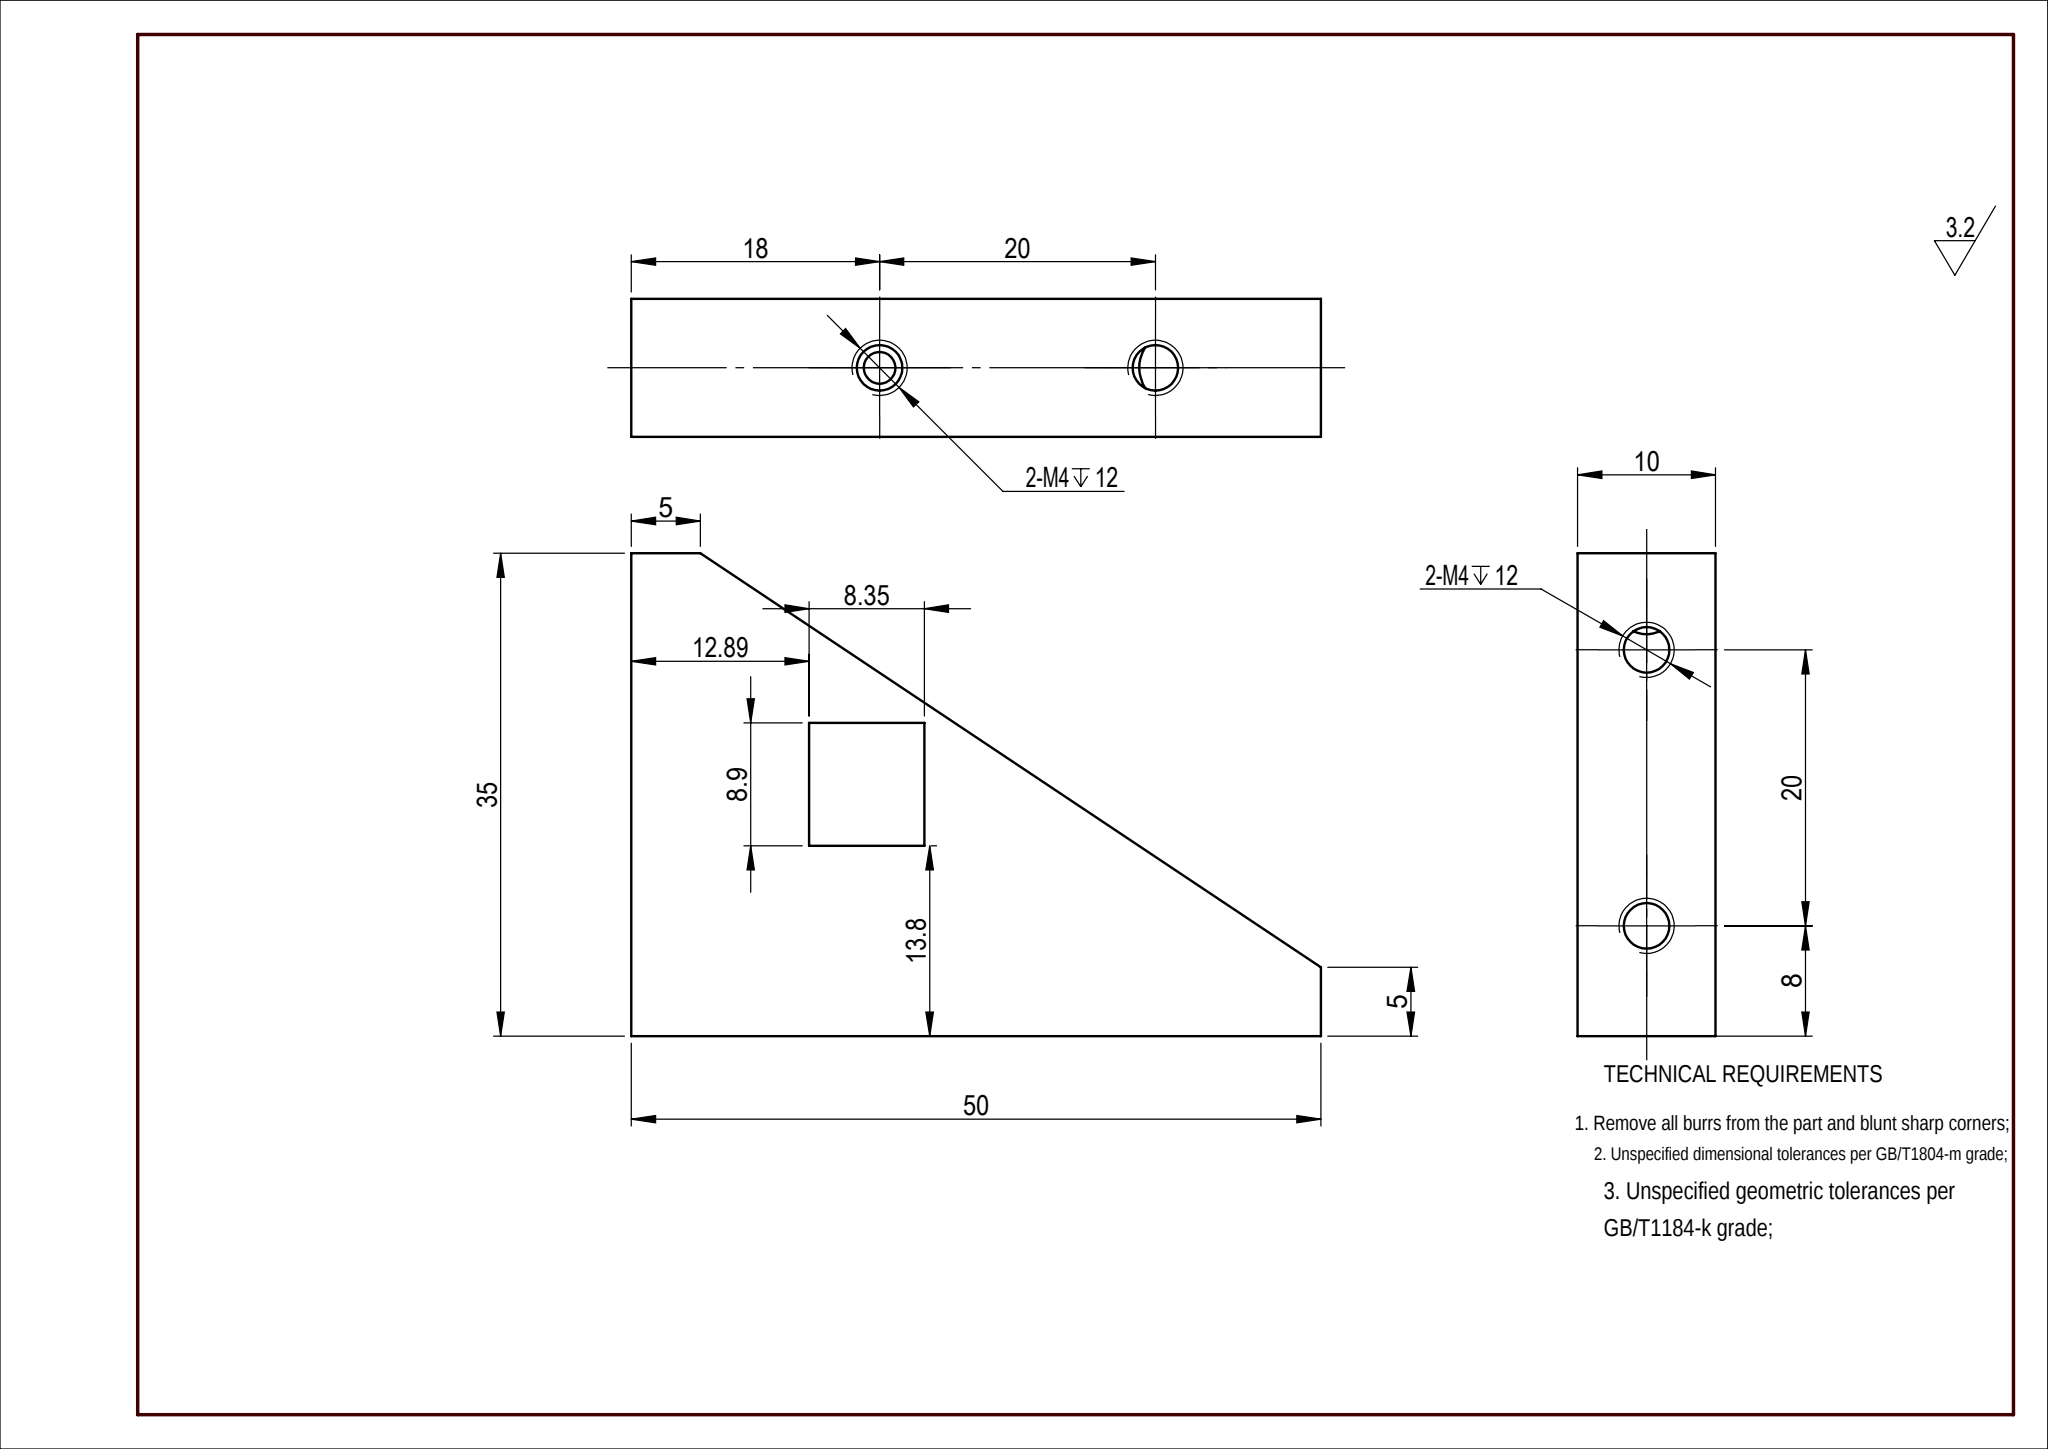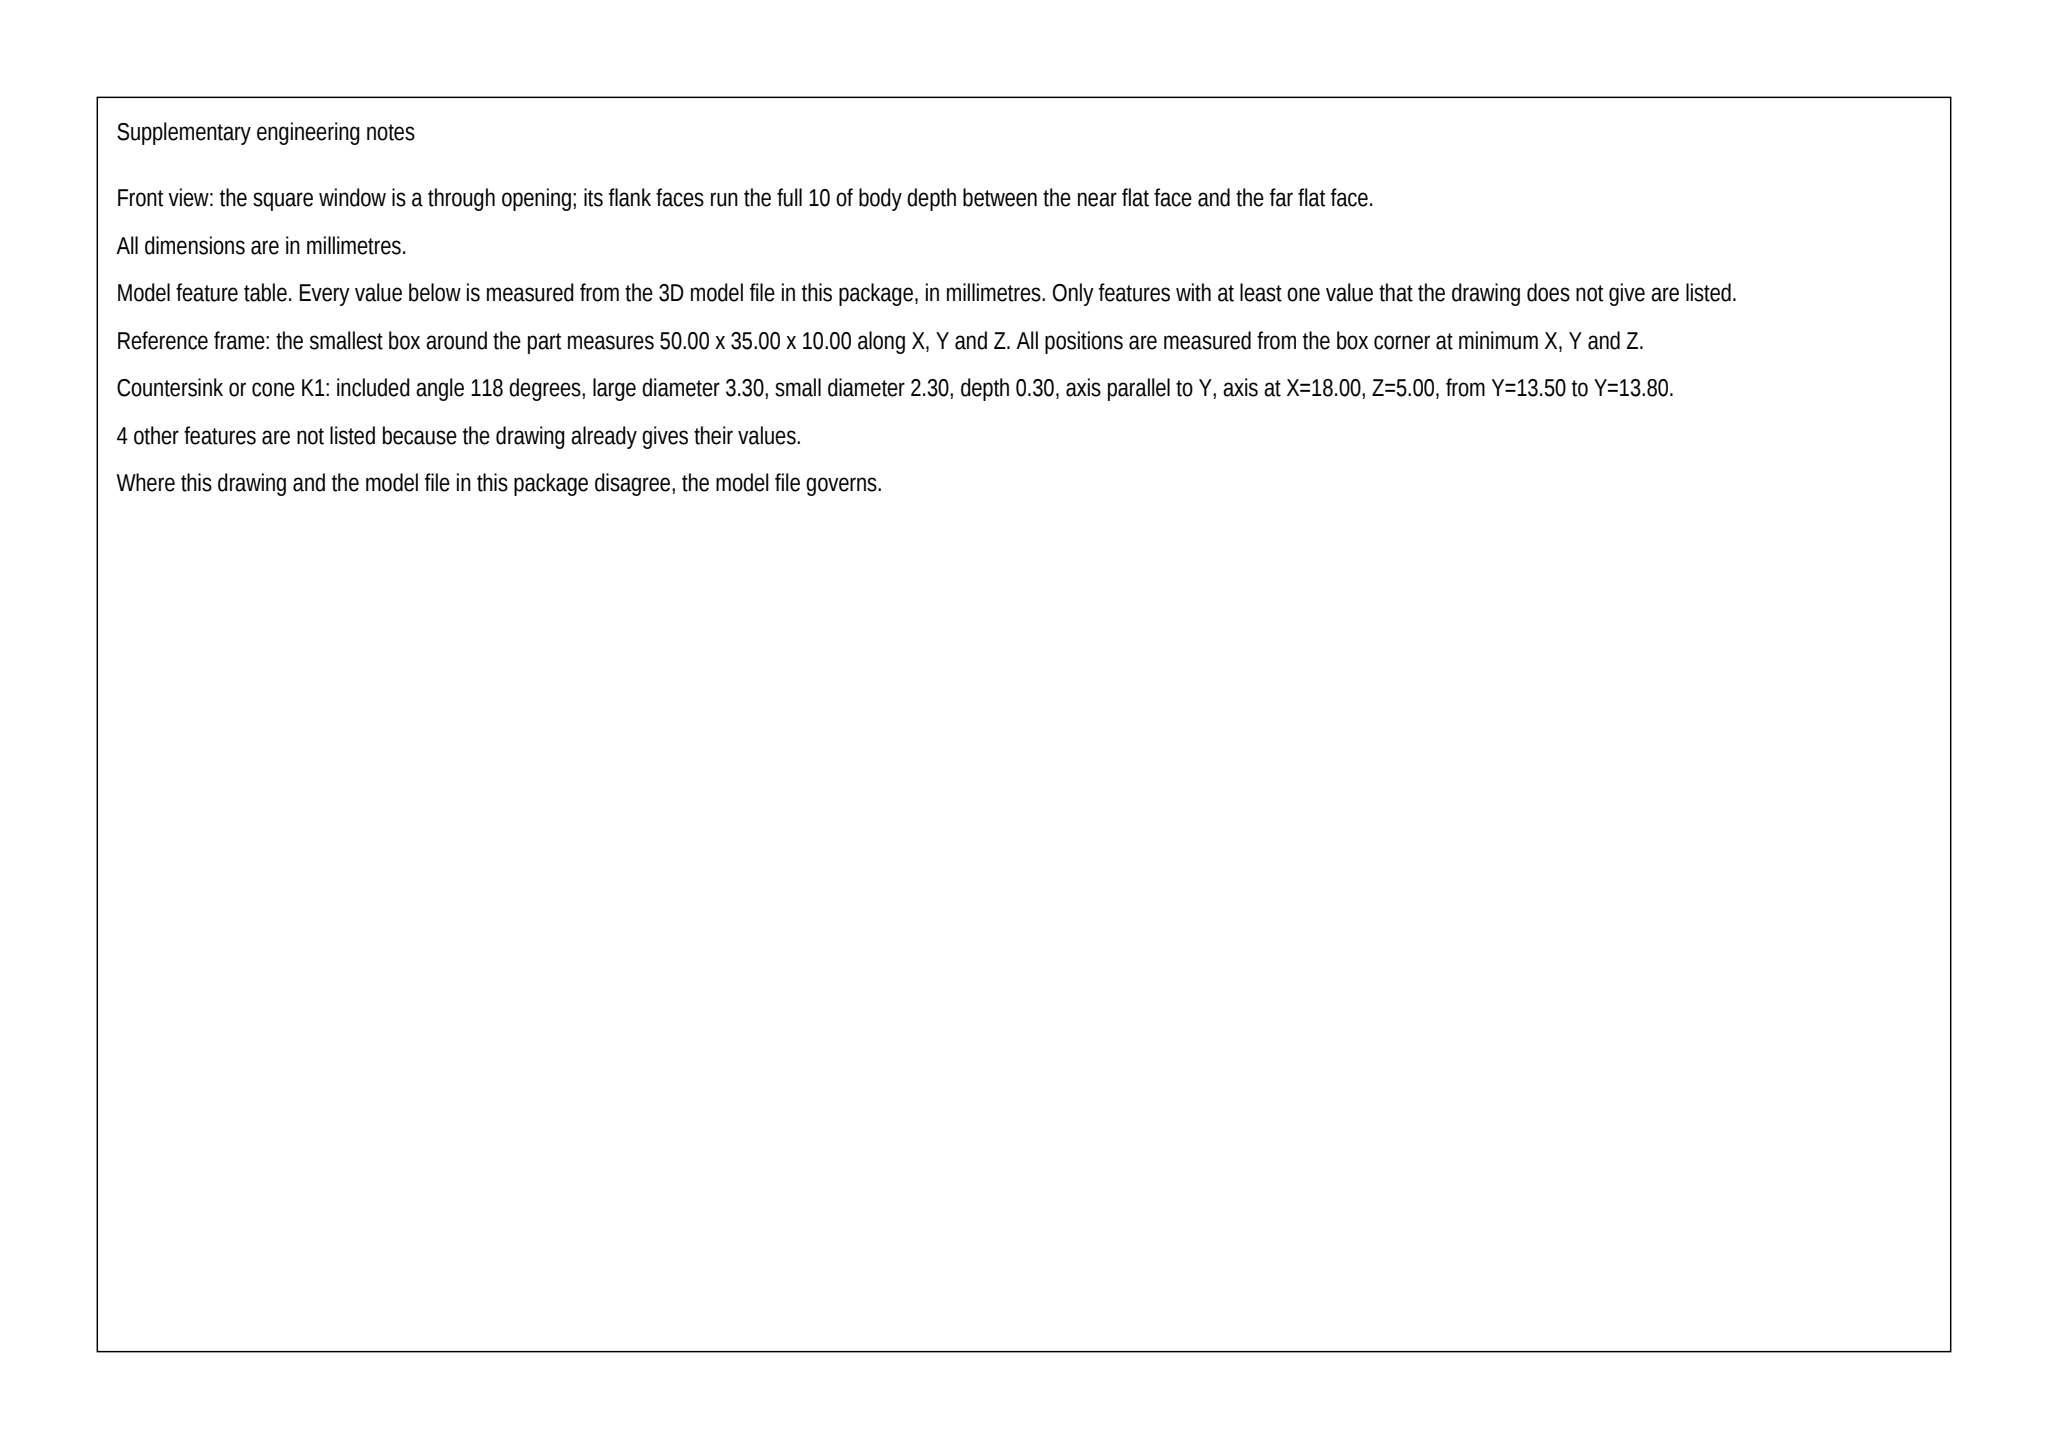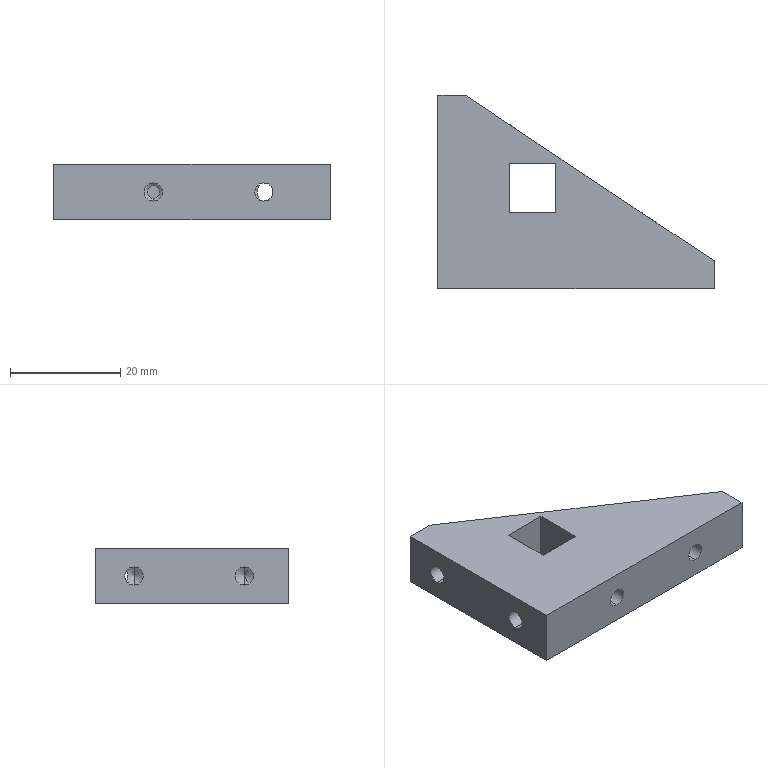Part | SolidWorks | mm | 1 solid | 26 faces | box 50 x 35 x 10 mm | volume 9542 mm3 | plane 11 | cylinder 8 | cone 7 | commonest cylinder face diameters 3.3 x8
build123d program:
from build123d import *

# Parameters (mm, degrees)
BOSS_EXTRUDE1_DEPTH   = 5
M4_TAPPED_HOLE1_D     = 3.3
M4_TAPPED_HOLE1_DEPTH = 13.5
M4_TAPPED_HOLE1_TIP   = 0.9914
M4_TAPPED_HOLE2_D     = 3.3
M4_TAPPED_HOLE2_DEPTH = 13.5
M4_TAPPED_HOLE2_TIP   = 0.9914
SKETCH6_W             = 8.348
SKETCH6_H             = 8.902
CUT_EXTRUDE1_DEPTH    = 22


with BuildPart() as part:
    # Sketch1 → Boss-Extrude1 (new, symmetric)
    with BuildSketch(Plane.XY):
        Polygon((0, 0), (0, 35), (5, 35), (50, 5), (50, 0), align=None)
    extrude(amount=BOSS_EXTRUDE1_DEPTH, both=True)

    # M4 Tapped Hole1
    with Locations(Plane.ZY):
        with Locations((0, 8), (0, 28)):
            Hole(M4_TAPPED_HOLE1_D / 2, depth=M4_TAPPED_HOLE1_DEPTH)
            with Locations((0, 0, -(M4_TAPPED_HOLE1_DEPTH + M4_TAPPED_HOLE1_TIP / 2))):  # 118° drill point
                Cone(0, M4_TAPPED_HOLE1_D / 2, M4_TAPPED_HOLE1_TIP, mode=Mode.SUBTRACT)

    # M4 Tapped Hole2
    with Locations(Plane.XZ):
        with Locations((18, 0), (38, 0)):
            Hole(M4_TAPPED_HOLE2_D / 2, depth=M4_TAPPED_HOLE2_DEPTH)
            with Locations((0, 0, -(M4_TAPPED_HOLE2_DEPTH + M4_TAPPED_HOLE2_TIP / 2))):  # 118° drill point
                Cone(0, M4_TAPPED_HOLE2_D / 2, M4_TAPPED_HOLE2_TIP, mode=Mode.SUBTRACT)

    # Sketch6 → Cut-Extrude1 (cut)
    with BuildSketch(Plane(origin=(0, 0, -5), x_dir=(-1, 0, 0), z_dir=(0, 0, -1))):
        with Locations((-17.067, 18.252)):
            Rectangle(SKETCH6_W, SKETCH6_H)
    extrude(amount=-CUT_EXTRUDE1_DEPTH, mode=Mode.SUBTRACT)


solid = part.part
STEP:
#1=CARTESIAN_POINT('',(18.,13.5,1.65));
#2=VERTEX_POINT('',#1);
#3=CARTESIAN_POINT('',(18.,13.5,-1.65));
#4=VERTEX_POINT('',#3);
#5=CARTESIAN_POINT('',(18.,13.5,0.));
#6=DIRECTION('',(0.,-1.,0.));
#7=DIRECTION('',(0.,0.,-1.));
#8=AXIS2_PLACEMENT_3D('',#5,#6,#7);
#9=CIRCLE('',#8,1.65);
#10=EDGE_CURVE('',#2,#4,#9,.T.);
#11=ORIENTED_EDGE('',*,*,#10,.F.);
#12=CARTESIAN_POINT('',(18.,-0.,1.65));
#13=VERTEX_POINT('',#12);
#14=CARTESIAN_POINT('',(18.,0.,1.65));
#15=DIRECTION('',(0.,-1.,0.));
#16=VECTOR('',#15,1000.);
#17=LINE('',#14,#16);
#18=EDGE_CURVE('',#2,#13,#17,.T.);
#19=ORIENTED_EDGE('',*,*,#18,.T.);
#20=CARTESIAN_POINT('',(18.,-0.,-1.65));
#21=VERTEX_POINT('',#20);
#22=CARTESIAN_POINT('',(18.,-0.,0.));
#23=DIRECTION('',(0.,-1.,0.));
#24=DIRECTION('',(0.,0.,-1.));
#25=AXIS2_PLACEMENT_3D('',#22,#23,#24);
#26=CIRCLE('',#25,1.65);
#27=EDGE_CURVE('',#13,#21,#26,.T.);
#28=ORIENTED_EDGE('',*,*,#27,.T.);
#29=CARTESIAN_POINT('',(18.,0.,-1.65));
#30=DIRECTION('',(0.,-1.,0.));
#31=VECTOR('',#30,1000.);
#32=LINE('',#29,#31);
#33=EDGE_CURVE('',#4,#21,#32,.T.);
#34=ORIENTED_EDGE('',*,*,#33,.F.);
#35=EDGE_LOOP('',(#11,#19,#28,#34));
#36=FACE_OUTER_BOUND('',#35,.T.);
#37=CARTESIAN_POINT('',(18.,0.,0.));
#38=DIRECTION('',(0.,-1.,0.));
#39=DIRECTION('',(0.,0.,-1.));
#40=AXIS2_PLACEMENT_3D('',#37,#38,#39);
#41=CYLINDRICAL_SURFACE('',#40,1.65);
#42=ADVANCED_FACE('',(#36),#41,.F.);
#43=CARTESIAN_POINT('',(18.,13.801,-1.149));
#44=VERTEX_POINT('',#43);
#45=CARTESIAN_POINT('',(18.,13.801,1.149));
#46=VERTEX_POINT('',#45);
#47=CARTESIAN_POINT('',(18.,13.801,0.));
#48=DIRECTION('',(0.,1.,0.));
#49=DIRECTION('',(0.,0.,-1.));
#50=AXIS2_PLACEMENT_3D('',#47,#48,#49);
#51=CIRCLE('',#50,1.149);
#52=EDGE_CURVE('',#44,#46,#51,.T.);
#53=ORIENTED_EDGE('',*,*,#52,.T.);
#54=CARTESIAN_POINT('',(18.,13.5,1.65));
#55=DIRECTION('',(0.,-0.515,0.8572));
#56=VECTOR('',#55,1000.);
#57=LINE('',#54,#56);
#58=EDGE_CURVE('',#46,#2,#57,.T.);
#59=ORIENTED_EDGE('',*,*,#58,.T.);
#60=ORIENTED_EDGE('',*,*,#10,.T.);
#61=CARTESIAN_POINT('',(18.,13.5,-1.65));
#62=DIRECTION('',(0.,-0.515,-0.8572));
#63=VECTOR('',#62,1000.);
#64=LINE('',#61,#63);
#65=EDGE_CURVE('',#44,#4,#64,.T.);
#66=ORIENTED_EDGE('',*,*,#65,.F.);
#67=EDGE_LOOP('',(#53,#59,#60,#66));
#68=FACE_OUTER_BOUND('',#67,.T.);
#69=CARTESIAN_POINT('',(18.,13.5,0.));
#70=DIRECTION('',(0.,-1.,0.));
#71=DIRECTION('',(0.,0.,-1.));
#72=AXIS2_PLACEMENT_3D('',#69,#70,#71);
#73=CONICAL_SURFACE('',#72,1.65,1.03);
#74=ADVANCED_FACE('',(#68),#73,.F.);
#75=CARTESIAN_POINT('',(38.,13.,1.65));
#76=VERTEX_POINT('',#75);
#77=CARTESIAN_POINT('',(37.25,13.5,1.47));
#78=VERTEX_POINT('',#77);
#79=CARTESIAN_POINT('',(38.,13.,1.65));
#80=CARTESIAN_POINT('',(37.738,13.175,1.65));
#81=CARTESIAN_POINT('',(37.483,13.344,1.589));
#82=CARTESIAN_POINT('',(37.25,13.5,1.47));
#83=(BOUNDED_CURVE()B_SPLINE_CURVE(3,(#79,#80,#81,#82),.UNSPECIFIED.,.F.,.F.)B_SPLINE_CURVE_WITH_KNOTS((4,4),(1.571,2.043),.UNSPECIFIED.)CURVE()GEOMETRIC_REPRESENTATION_ITEM()RATIONAL_B_SPLINE_CURVE((1.,0.9815,0.9815,1.))REPRESENTATION_ITEM(''));
#84=EDGE_CURVE('',#76,#78,#83,.T.);
#85=ORIENTED_EDGE('',*,*,#84,.F.);
#86=CARTESIAN_POINT('',(38.,-0.,1.65));
#87=VERTEX_POINT('',#86);
#88=CARTESIAN_POINT('',(38.,0.,1.65));
#89=DIRECTION('',(0.,-1.,0.));
#90=VECTOR('',#89,1000.);
#91=LINE('',#88,#90);
#92=EDGE_CURVE('',#76,#87,#91,.T.);
#93=ORIENTED_EDGE('',*,*,#92,.T.);
#94=CARTESIAN_POINT('',(38.,-0.,-1.65));
#95=VERTEX_POINT('',#94);
#96=CARTESIAN_POINT('',(38.,-0.,0.));
#97=DIRECTION('',(0.,-1.,0.));
#98=DIRECTION('',(0.,0.,-1.));
#99=AXIS2_PLACEMENT_3D('',#96,#97,#98);
#100=CIRCLE('',#99,1.65);
#101=EDGE_CURVE('',#87,#95,#100,.T.);
#102=ORIENTED_EDGE('',*,*,#101,.T.);
#103=CARTESIAN_POINT('',(38.,13.,-1.65));
#104=VERTEX_POINT('',#103);
#105=CARTESIAN_POINT('',(38.,0.,-1.65));
#106=DIRECTION('',(0.,-1.,0.));
#107=VECTOR('',#106,1000.);
#108=LINE('',#105,#107);
#109=EDGE_CURVE('',#104,#95,#108,.T.);
#110=ORIENTED_EDGE('',*,*,#109,.F.);
#111=CARTESIAN_POINT('',(37.25,13.5,-1.47));
#112=VERTEX_POINT('',#111);
#113=CARTESIAN_POINT('',(37.25,13.5,-1.47));
#114=CARTESIAN_POINT('',(37.483,13.344,-1.589));
#115=CARTESIAN_POINT('',(37.738,13.175,-1.65));
#116=CARTESIAN_POINT('',(38.,13.,-1.65));
#117=(BOUNDED_CURVE()B_SPLINE_CURVE(3,(#113,#114,#115,#116),.UNSPECIFIED.,.F.,.F.)B_SPLINE_CURVE_WITH_KNOTS((4,4),(4.241,4.712),.UNSPECIFIED.)CURVE()GEOMETRIC_REPRESENTATION_ITEM()RATIONAL_B_SPLINE_CURVE((1.,0.9815,0.9815,1.))REPRESENTATION_ITEM(''));
#118=EDGE_CURVE('',#112,#104,#117,.T.);
#119=ORIENTED_EDGE('',*,*,#118,.F.);
#120=CARTESIAN_POINT('',(38.,13.5,0.));
#121=DIRECTION('',(0.,-1.,0.));
#122=DIRECTION('',(0.,0.,-1.));
#123=AXIS2_PLACEMENT_3D('',#120,#121,#122);
#124=CIRCLE('',#123,1.65);
#125=EDGE_CURVE('',#78,#112,#124,.T.);
#126=ORIENTED_EDGE('',*,*,#125,.F.);
#127=EDGE_LOOP('',(#85,#93,#102,#110,#119,#126));
#128=FACE_OUTER_BOUND('',#127,.T.);
#129=CARTESIAN_POINT('',(38.,0.,0.));
#130=DIRECTION('',(0.,-1.,0.));
#131=DIRECTION('',(0.,0.,-1.));
#132=AXIS2_PLACEMENT_3D('',#129,#130,#131);
#133=CYLINDRICAL_SURFACE('',#132,1.65);
#134=ADVANCED_FACE('',(#128),#133,.F.);
#135=CARTESIAN_POINT('',(13.5,8.,-1.65));
#136=VERTEX_POINT('',#135);
#137=CARTESIAN_POINT('',(13.5,8.,1.65));
#138=VERTEX_POINT('',#137);
#139=CARTESIAN_POINT('',(13.5,8.,0.));
#140=DIRECTION('',(-1.,0.,0.));
#141=DIRECTION('',(0.,0.,1.));
#142=AXIS2_PLACEMENT_3D('',#139,#140,#141);
#143=CIRCLE('',#142,1.65);
#144=EDGE_CURVE('',#136,#138,#143,.T.);
#145=ORIENTED_EDGE('',*,*,#144,.F.);
#146=CARTESIAN_POINT('',(-0.,8.,-1.65));
#147=VERTEX_POINT('',#146);
#148=CARTESIAN_POINT('',(0.,8.,-1.65));
#149=DIRECTION('',(-1.,0.,0.));
#150=VECTOR('',#149,1000.);
#151=LINE('',#148,#150);
#152=EDGE_CURVE('',#136,#147,#151,.T.);
#153=ORIENTED_EDGE('',*,*,#152,.T.);
#154=CARTESIAN_POINT('',(-0.,8.,1.65));
#155=VERTEX_POINT('',#154);
#156=CARTESIAN_POINT('',(-0.,8.,0.));
#157=DIRECTION('',(-1.,0.,0.));
#158=DIRECTION('',(0.,0.,1.));
#159=AXIS2_PLACEMENT_3D('',#156,#157,#158);
#160=CIRCLE('',#159,1.65);
#161=EDGE_CURVE('',#147,#155,#160,.T.);
#162=ORIENTED_EDGE('',*,*,#161,.T.);
#163=CARTESIAN_POINT('',(0.,8.,1.65));
#164=DIRECTION('',(-1.,0.,0.));
#165=VECTOR('',#164,1000.);
#166=LINE('',#163,#165);
#167=EDGE_CURVE('',#138,#155,#166,.T.);
#168=ORIENTED_EDGE('',*,*,#167,.F.);
#169=EDGE_LOOP('',(#145,#153,#162,#168));
#170=FACE_OUTER_BOUND('',#169,.T.);
#171=CARTESIAN_POINT('',(0.,8.,0.));
#172=DIRECTION('',(-1.,0.,0.));
#173=DIRECTION('',(0.,0.,1.));
#174=AXIS2_PLACEMENT_3D('',#171,#172,#173);
#175=CYLINDRICAL_SURFACE('',#174,1.65);
#176=ADVANCED_FACE('',(#170),#175,.F.);
#177=CARTESIAN_POINT('',(14.491,8.,0.));
#178=VERTEX_POINT('',#177);
#179=CARTESIAN_POINT('',(13.5,8.,1.65));
#180=DIRECTION('',(-0.515,0.,0.8572));
#181=VECTOR('',#180,1000.);
#182=LINE('',#179,#181);
#183=EDGE_CURVE('',#178,#138,#182,.T.);
#184=ORIENTED_EDGE('',*,*,#183,.F.);
#185=CARTESIAN_POINT('',(13.5,8.,-1.65));
#186=DIRECTION('',(-0.515,0.,-0.8572));
#187=VECTOR('',#186,1000.);
#188=LINE('',#185,#187);
#189=EDGE_CURVE('',#178,#136,#188,.T.);
#190=ORIENTED_EDGE('',*,*,#189,.T.);
#191=ORIENTED_EDGE('',*,*,#144,.T.);
#192=EDGE_LOOP('',(#184,#190,#191));
#193=FACE_OUTER_BOUND('',#192,.T.);
#194=CARTESIAN_POINT('',(13.5,8.,0.));
#195=DIRECTION('',(-1.,0.,0.));
#196=DIRECTION('',(0.,0.,1.));
#197=AXIS2_PLACEMENT_3D('',#194,#195,#196);
#198=CONICAL_SURFACE('',#197,1.65,1.03);
#199=ADVANCED_FACE('',(#193),#198,.F.);
#200=CARTESIAN_POINT('',(14.491,28.,0.));
#201=VERTEX_POINT('',#200);
#202=CARTESIAN_POINT('',(13.5,28.,1.65));
#203=VERTEX_POINT('',#202);
#204=CARTESIAN_POINT('',(13.5,28.,1.65));
#205=DIRECTION('',(-0.515,0.,0.8572));
#206=VECTOR('',#205,1000.);
#207=LINE('',#204,#206);
#208=EDGE_CURVE('',#201,#203,#207,.T.);
#209=ORIENTED_EDGE('',*,*,#208,.F.);
#210=CARTESIAN_POINT('',(13.5,28.,-1.65));
#211=VERTEX_POINT('',#210);
#212=CARTESIAN_POINT('',(13.5,28.,-1.65));
#213=DIRECTION('',(-0.515,0.,-0.8572));
#214=VECTOR('',#213,1000.);
#215=LINE('',#212,#214);
#216=EDGE_CURVE('',#201,#211,#215,.T.);
#217=ORIENTED_EDGE('',*,*,#216,.T.);
#218=CARTESIAN_POINT('',(13.5,28.,0.));
#219=DIRECTION('',(-1.,0.,0.));
#220=DIRECTION('',(0.,0.,1.));
#221=AXIS2_PLACEMENT_3D('',#218,#219,#220);
#222=CIRCLE('',#221,1.65);
#223=EDGE_CURVE('',#211,#203,#222,.T.);
#224=ORIENTED_EDGE('',*,*,#223,.T.);
#225=EDGE_LOOP('',(#209,#217,#224));
#226=FACE_OUTER_BOUND('',#225,.T.);
#227=CARTESIAN_POINT('',(13.5,28.,0.));
#228=DIRECTION('',(-1.,0.,0.));
#229=DIRECTION('',(0.,0.,1.));
#230=AXIS2_PLACEMENT_3D('',#227,#228,#229);
#231=CONICAL_SURFACE('',#230,1.65,1.03);
#232=ADVANCED_FACE('',(#226),#231,.F.);
#233=ORIENTED_EDGE('',*,*,#223,.F.);
#234=CARTESIAN_POINT('',(-0.,28.,-1.65));
#235=VERTEX_POINT('',#234);
#236=CARTESIAN_POINT('',(0.,28.,-1.65));
#237=DIRECTION('',(-1.,0.,0.));
#238=VECTOR('',#237,1000.);
#239=LINE('',#236,#238);
#240=EDGE_CURVE('',#211,#235,#239,.T.);
#241=ORIENTED_EDGE('',*,*,#240,.T.);
#242=CARTESIAN_POINT('',(-0.,28.,1.65));
#243=VERTEX_POINT('',#242);
#244=CARTESIAN_POINT('',(-0.,28.,0.));
#245=DIRECTION('',(-1.,0.,0.));
#246=DIRECTION('',(0.,0.,1.));
#247=AXIS2_PLACEMENT_3D('',#244,#245,#246);
#248=CIRCLE('',#247,1.65);
#249=EDGE_CURVE('',#235,#243,#248,.T.);
#250=ORIENTED_EDGE('',*,*,#249,.T.);
#251=CARTESIAN_POINT('',(0.,28.,1.65));
#252=DIRECTION('',(-1.,0.,0.));
#253=VECTOR('',#252,1000.);
#254=LINE('',#251,#253);
#255=EDGE_CURVE('',#203,#243,#254,.T.);
#256=ORIENTED_EDGE('',*,*,#255,.F.);
#257=EDGE_LOOP('',(#233,#241,#250,#256));
#258=FACE_OUTER_BOUND('',#257,.T.);
#259=CARTESIAN_POINT('',(0.,28.,0.));
#260=DIRECTION('',(-1.,0.,0.));
#261=DIRECTION('',(0.,0.,1.));
#262=AXIS2_PLACEMENT_3D('',#259,#260,#261);
#263=CYLINDRICAL_SURFACE('',#262,1.65);
#264=ADVANCED_FACE('',(#258),#263,.F.);
#265=CARTESIAN_POINT('',(18.,-0.,0.));
#266=DIRECTION('',(0.,-1.,0.));
#267=DIRECTION('',(0.,0.,-1.));
#268=AXIS2_PLACEMENT_3D('',#265,#266,#267);
#269=CIRCLE('',#268,1.65);
#270=EDGE_CURVE('',#21,#13,#269,.T.);
#271=ORIENTED_EDGE('',*,*,#270,.F.);
#272=ORIENTED_EDGE('',*,*,#27,.F.);
#273=EDGE_LOOP('',(#271,#272));
#274=FACE_BOUND('',#273,.T.);
#275=CARTESIAN_POINT('',(38.,-0.,0.));
#276=DIRECTION('',(0.,-1.,0.));
#277=DIRECTION('',(0.,0.,-1.));
#278=AXIS2_PLACEMENT_3D('',#275,#276,#277);
#279=CIRCLE('',#278,1.65);
#280=EDGE_CURVE('',#95,#87,#279,.T.);
#281=ORIENTED_EDGE('',*,*,#280,.F.);
#282=ORIENTED_EDGE('',*,*,#101,.F.);
#283=EDGE_LOOP('',(#281,#282));
#284=FACE_BOUND('',#283,.T.);
#285=CARTESIAN_POINT('',(0.,0.,-5.));
#286=VERTEX_POINT('',#285);
#287=CARTESIAN_POINT('',(50.,0.,-5.));
#288=VERTEX_POINT('',#287);
#289=CARTESIAN_POINT('',(50.,0.,-5.));
#290=DIRECTION('',(1.,0.,0.));
#291=VECTOR('',#290,1000.);
#292=LINE('',#289,#291);
#293=EDGE_CURVE('',#286,#288,#292,.T.);
#294=ORIENTED_EDGE('',*,*,#293,.T.);
#295=CARTESIAN_POINT('',(50.,0.,5.));
#296=VERTEX_POINT('',#295);
#297=CARTESIAN_POINT('',(50.,0.,5.));
#298=DIRECTION('',(0.,0.,-1.));
#299=VECTOR('',#298,1000.);
#300=LINE('',#297,#299);
#301=EDGE_CURVE('',#296,#288,#300,.T.);
#302=ORIENTED_EDGE('',*,*,#301,.F.);
#303=CARTESIAN_POINT('',(0.,0.,5.));
#304=VERTEX_POINT('',#303);
#305=CARTESIAN_POINT('',(50.,0.,5.));
#306=DIRECTION('',(1.,0.,0.));
#307=VECTOR('',#306,1000.);
#308=LINE('',#305,#307);
#309=EDGE_CURVE('',#304,#296,#308,.T.);
#310=ORIENTED_EDGE('',*,*,#309,.F.);
#311=CARTESIAN_POINT('',(0.,0.,5.));
#312=DIRECTION('',(0.,0.,-1.));
#313=VECTOR('',#312,1000.);
#314=LINE('',#311,#313);
#315=EDGE_CURVE('',#304,#286,#314,.T.);
#316=ORIENTED_EDGE('',*,*,#315,.T.);
#317=EDGE_LOOP('',(#294,#302,#310,#316));
#318=FACE_OUTER_BOUND('',#317,.T.);
#319=CARTESIAN_POINT('',(50.,0.,5.));
#320=DIRECTION('',(-0.,1.,0.));
#321=DIRECTION('',(-1.,-0.,0.));
#322=AXIS2_PLACEMENT_3D('',#319,#320,#321);
#323=PLANE('',#322);
#324=ADVANCED_FACE('',(#274,#284,#318),#323,.F.);
#325=CARTESIAN_POINT('',(50.,5.,-5.));
#326=VERTEX_POINT('',#325);
#327=CARTESIAN_POINT('',(50.,5.,-5.));
#328=DIRECTION('',(0.,1.,0.));
#329=VECTOR('',#328,1000.);
#330=LINE('',#327,#329);
#331=EDGE_CURVE('',#288,#326,#330,.T.);
#332=ORIENTED_EDGE('',*,*,#331,.T.);
#333=CARTESIAN_POINT('',(50.,5.,5.));
#334=VERTEX_POINT('',#333);
#335=CARTESIAN_POINT('',(50.,5.,5.));
#336=DIRECTION('',(0.,0.,-1.));
#337=VECTOR('',#336,1000.);
#338=LINE('',#335,#337);
#339=EDGE_CURVE('',#334,#326,#338,.T.);
#340=ORIENTED_EDGE('',*,*,#339,.F.);
#341=CARTESIAN_POINT('',(50.,5.,5.));
#342=DIRECTION('',(0.,1.,0.));
#343=VECTOR('',#342,1000.);
#344=LINE('',#341,#343);
#345=EDGE_CURVE('',#296,#334,#344,.T.);
#346=ORIENTED_EDGE('',*,*,#345,.F.);
#347=ORIENTED_EDGE('',*,*,#301,.T.);
#348=EDGE_LOOP('',(#332,#340,#346,#347));
#349=FACE_OUTER_BOUND('',#348,.T.);
#350=CARTESIAN_POINT('',(50.,5.,5.));
#351=DIRECTION('',(-1.,0.,0.));
#352=DIRECTION('',(0.,0.,1.));
#353=AXIS2_PLACEMENT_3D('',#350,#351,#352);
#354=PLANE('',#353);
#355=ADVANCED_FACE('',(#349),#354,.F.);
#356=CARTESIAN_POINT('',(37.25,13.5,1.47));
#357=CARTESIAN_POINT('',(37.126,13.583,1.251));
#358=CARTESIAN_POINT('',(37.02,13.653,1.022));
#359=CARTESIAN_POINT('',(36.905,13.73,0.6503));
#360=CARTESIAN_POINT('',(36.875,13.75,0.5222));
#361=CARTESIAN_POINT('',(36.834,13.777,0.2644));
#362=CARTESIAN_POINT('',(36.823,13.784,0.1338));
#363=CARTESIAN_POINT('',(36.823,13.785,-0.2638));
#364=CARTESIAN_POINT('',(36.866,13.756,-0.5233));
#365=CARTESIAN_POINT('',(37.019,13.654,-1.021));
#366=CARTESIAN_POINT('',(37.126,13.583,-1.251));
#367=CARTESIAN_POINT('',(37.25,13.5,-1.47));
#368=B_SPLINE_CURVE_WITH_KNOTS('',3,(#356,#357,#358,#359,#360,#361,#362,#363,#364,#365,#366,#367),.UNSPECIFIED.,.F.,.F.,(4,2,2,2,2,4),(0.00000063,0.0007877,0.001181,0.001575,0.002362,0.003149),.UNSPECIFIED.);
#369=EDGE_CURVE('',#78,#112,#368,.T.);
#370=ORIENTED_EDGE('',*,*,#369,.T.);
#371=ORIENTED_EDGE('',*,*,#118,.T.);
#372=CARTESIAN_POINT('',(38.,13.,-1.65));
#373=CARTESIAN_POINT('',(41.3,10.8,-1.65));
#374=CARTESIAN_POINT('',(41.3,10.8,1.65));
#375=CARTESIAN_POINT('',(38.,13.,1.65));
#376=(BOUNDED_CURVE()B_SPLINE_CURVE(3,(#372,#373,#374,#375),.UNSPECIFIED.,.F.,.F.)B_SPLINE_CURVE_WITH_KNOTS((4,4),(4.712,7.854),.UNSPECIFIED.)CURVE()GEOMETRIC_REPRESENTATION_ITEM()RATIONAL_B_SPLINE_CURVE((1.,0.3333,0.3333,1.))REPRESENTATION_ITEM(''));
#377=EDGE_CURVE('',#104,#76,#376,.T.);
#378=ORIENTED_EDGE('',*,*,#377,.T.);
#379=ORIENTED_EDGE('',*,*,#84,.T.);
#380=EDGE_LOOP('',(#370,#371,#378,#379));
#381=FACE_BOUND('',#380,.T.);
#382=CARTESIAN_POINT('',(13.5,29.333,-0.972));
#383=VERTEX_POINT('',#382);
#384=CARTESIAN_POINT('',(13.5,29.333,0.972));
#385=VERTEX_POINT('',#384);
#386=CARTESIAN_POINT('',(13.5,29.333,-0.972));
#387=CARTESIAN_POINT('',(13.578,29.281,-0.823));
#388=CARTESIAN_POINT('',(13.652,29.232,-0.6716));
#389=CARTESIAN_POINT('',(13.772,29.152,-0.3521));
#390=CARTESIAN_POINT('',(13.817,29.122,-0.1794));
#391=CARTESIAN_POINT('',(13.818,29.122,0.08435));
#392=CARTESIAN_POINT('',(13.807,29.129,0.1736));
#393=CARTESIAN_POINT('',(13.77,29.153,0.344));
#394=CARTESIAN_POINT('',(13.744,29.171,0.4269));
#395=CARTESIAN_POINT('',(13.653,29.231,0.6696));
#396=CARTESIAN_POINT('',(13.578,29.281,0.822));
#397=CARTESIAN_POINT('',(13.5,29.333,0.972));
#398=B_SPLINE_CURVE_WITH_KNOTS('',3,(#386,#387,#388,#389,#390,#391,#392,#393,#394,#395,#396,#397),.UNSPECIFIED.,.F.,.F.,(4,2,2,2,2,4),(0.00000045,0.0005259,0.001051,0.001314,0.001577,0.002102),.UNSPECIFIED.);
#399=EDGE_CURVE('',#383,#385,#398,.T.);
#400=ORIENTED_EDGE('',*,*,#399,.T.);
#401=CARTESIAN_POINT('',(13.5,29.333,0.972));
#402=CARTESIAN_POINT('',(12.843,29.771,0.3715));
#403=CARTESIAN_POINT('',(12.843,29.771,-0.3715));
#404=CARTESIAN_POINT('',(13.5,29.333,-0.972));
#405=(BOUNDED_CURVE()B_SPLINE_CURVE(3,(#401,#402,#403,#404),.UNSPECIFIED.,.F.,.F.)B_SPLINE_CURVE_WITH_KNOTS((4,4),(5.653,6.913),.UNSPECIFIED.)CURVE()GEOMETRIC_REPRESENTATION_ITEM()RATIONAL_B_SPLINE_CURVE((1.,0.8721,0.8721,1.))REPRESENTATION_ITEM(''));
#406=EDGE_CURVE('',#385,#383,#405,.T.);
#407=ORIENTED_EDGE('',*,*,#406,.T.);
#408=EDGE_LOOP('',(#400,#407));
#409=FACE_BOUND('',#408,.T.);
#410=CARTESIAN_POINT('',(5.,35.,-5.));
#411=VERTEX_POINT('',#410);
#412=CARTESIAN_POINT('',(5.,35.,-5.));
#413=DIRECTION('',(-0.8321,0.5547,0.));
#414=VECTOR('',#413,1000.);
#415=LINE('',#412,#414);
#416=EDGE_CURVE('',#326,#411,#415,.T.);
#417=ORIENTED_EDGE('',*,*,#416,.T.);
#418=CARTESIAN_POINT('',(5.,35.,5.));
#419=VERTEX_POINT('',#418);
#420=CARTESIAN_POINT('',(5.,35.,5.));
#421=DIRECTION('',(0.,0.,-1.));
#422=VECTOR('',#421,1000.);
#423=LINE('',#420,#422);
#424=EDGE_CURVE('',#419,#411,#423,.T.);
#425=ORIENTED_EDGE('',*,*,#424,.F.);
#426=CARTESIAN_POINT('',(5.,35.,5.));
#427=DIRECTION('',(-0.8321,0.5547,0.));
#428=VECTOR('',#427,1000.);
#429=LINE('',#426,#428);
#430=EDGE_CURVE('',#334,#419,#429,.T.);
#431=ORIENTED_EDGE('',*,*,#430,.F.);
#432=ORIENTED_EDGE('',*,*,#339,.T.);
#433=EDGE_LOOP('',(#417,#425,#431,#432));
#434=FACE_OUTER_BOUND('',#433,.T.);
#435=CARTESIAN_POINT('',(5.,35.,5.));
#436=DIRECTION('',(-0.5547,-0.8321,0.));
#437=DIRECTION('',(0.8321,-0.5547,0.));
#438=AXIS2_PLACEMENT_3D('',#435,#436,#437);
#439=PLANE('',#438);
#440=ADVANCED_FACE('',(#381,#409,#434),#439,.F.);
#441=CARTESIAN_POINT('',(0.,35.,-5.));
#442=VERTEX_POINT('',#441);
#443=CARTESIAN_POINT('',(0.,35.,-5.));
#444=DIRECTION('',(-1.,0.,0.));
#445=VECTOR('',#444,1000.);
#446=LINE('',#443,#445);
#447=EDGE_CURVE('',#411,#442,#446,.T.);
#448=ORIENTED_EDGE('',*,*,#447,.T.);
#449=CARTESIAN_POINT('',(0.,35.,5.));
#450=VERTEX_POINT('',#449);
#451=CARTESIAN_POINT('',(0.,35.,5.));
#452=DIRECTION('',(0.,0.,-1.));
#453=VECTOR('',#452,1000.);
#454=LINE('',#451,#453);
#455=EDGE_CURVE('',#450,#442,#454,.T.);
#456=ORIENTED_EDGE('',*,*,#455,.F.);
#457=CARTESIAN_POINT('',(0.,35.,5.));
#458=DIRECTION('',(-1.,0.,0.));
#459=VECTOR('',#458,1000.);
#460=LINE('',#457,#459);
#461=EDGE_CURVE('',#419,#450,#460,.T.);
#462=ORIENTED_EDGE('',*,*,#461,.F.);
#463=ORIENTED_EDGE('',*,*,#424,.T.);
#464=EDGE_LOOP('',(#448,#456,#462,#463));
#465=FACE_OUTER_BOUND('',#464,.T.);
#466=CARTESIAN_POINT('',(0.,35.,5.));
#467=DIRECTION('',(0.,-1.,0.));
#468=DIRECTION('',(0.,0.,-1.));
#469=AXIS2_PLACEMENT_3D('',#466,#467,#468);
#470=PLANE('',#469);
#471=ADVANCED_FACE('',(#465),#470,.F.);
#472=CARTESIAN_POINT('',(-0.,8.,0.));
#473=DIRECTION('',(-1.,0.,0.));
#474=DIRECTION('',(0.,0.,1.));
#475=AXIS2_PLACEMENT_3D('',#472,#473,#474);
#476=CIRCLE('',#475,1.65);
#477=EDGE_CURVE('',#155,#147,#476,.T.);
#478=ORIENTED_EDGE('',*,*,#477,.F.);
#479=ORIENTED_EDGE('',*,*,#161,.F.);
#480=EDGE_LOOP('',(#478,#479));
#481=FACE_BOUND('',#480,.T.);
#482=CARTESIAN_POINT('',(-0.,28.,0.));
#483=DIRECTION('',(-1.,0.,0.));
#484=DIRECTION('',(0.,0.,1.));
#485=AXIS2_PLACEMENT_3D('',#482,#483,#484);
#486=CIRCLE('',#485,1.65);
#487=EDGE_CURVE('',#243,#235,#486,.T.);
#488=ORIENTED_EDGE('',*,*,#487,.F.);
#489=ORIENTED_EDGE('',*,*,#249,.F.);
#490=EDGE_LOOP('',(#488,#489));
#491=FACE_BOUND('',#490,.T.);
#492=CARTESIAN_POINT('',(0.,0.,-5.));
#493=DIRECTION('',(0.,-1.,0.));
#494=VECTOR('',#493,1000.);
#495=LINE('',#492,#494);
#496=EDGE_CURVE('',#442,#286,#495,.T.);
#497=ORIENTED_EDGE('',*,*,#496,.T.);
#498=ORIENTED_EDGE('',*,*,#315,.F.);
#499=CARTESIAN_POINT('',(0.,0.,5.));
#500=DIRECTION('',(0.,-1.,0.));
#501=VECTOR('',#500,1000.);
#502=LINE('',#499,#501);
#503=EDGE_CURVE('',#450,#304,#502,.T.);
#504=ORIENTED_EDGE('',*,*,#503,.F.);
#505=ORIENTED_EDGE('',*,*,#455,.T.);
#506=EDGE_LOOP('',(#497,#498,#504,#505));
#507=FACE_OUTER_BOUND('',#506,.T.);
#508=CARTESIAN_POINT('',(0.,0.,5.));
#509=DIRECTION('',(1.,0.,0.));
#510=DIRECTION('',(0.,0.,-1.));
#511=AXIS2_PLACEMENT_3D('',#508,#509,#510);
#512=PLANE('',#511);
#513=ADVANCED_FACE('',(#481,#491,#507),#512,.F.);
#514=CARTESIAN_POINT('',(12.893,22.703,5.));
#515=VERTEX_POINT('',#514);
#516=CARTESIAN_POINT('',(21.241,22.703,5.));
#517=VERTEX_POINT('',#516);
#518=CARTESIAN_POINT('',(0.,22.703,5.));
#519=DIRECTION('',(1.,0.,0.));
#520=VECTOR('',#519,1000.);
#521=LINE('',#518,#520);
#522=EDGE_CURVE('',#515,#517,#521,.T.);
#523=ORIENTED_EDGE('',*,*,#522,.T.);
#524=CARTESIAN_POINT('',(21.241,13.801,5.));
#525=VERTEX_POINT('',#524);
#526=CARTESIAN_POINT('',(21.241,0.,5.));
#527=DIRECTION('',(0.,-1.,0.));
#528=VECTOR('',#527,1000.);
#529=LINE('',#526,#528);
#530=EDGE_CURVE('',#517,#525,#529,.T.);
#531=ORIENTED_EDGE('',*,*,#530,.T.);
#532=CARTESIAN_POINT('',(12.893,13.801,5.));
#533=VERTEX_POINT('',#532);
#534=CARTESIAN_POINT('',(0.,13.801,5.));
#535=DIRECTION('',(-1.,0.,0.));
#536=VECTOR('',#535,1000.);
#537=LINE('',#534,#536);
#538=EDGE_CURVE('',#525,#533,#537,.T.);
#539=ORIENTED_EDGE('',*,*,#538,.T.);
#540=CARTESIAN_POINT('',(12.893,0.,5.));
#541=DIRECTION('',(0.,1.,0.));
#542=VECTOR('',#541,1000.);
#543=LINE('',#540,#542);
#544=EDGE_CURVE('',#533,#515,#543,.T.);
#545=ORIENTED_EDGE('',*,*,#544,.T.);
#546=EDGE_LOOP('',(#523,#531,#539,#545));
#547=FACE_BOUND('',#546,.T.);
#548=ORIENTED_EDGE('',*,*,#309,.T.);
#549=ORIENTED_EDGE('',*,*,#345,.T.);
#550=ORIENTED_EDGE('',*,*,#430,.T.);
#551=ORIENTED_EDGE('',*,*,#461,.T.);
#552=ORIENTED_EDGE('',*,*,#503,.T.);
#553=EDGE_LOOP('',(#548,#549,#550,#551,#552));
#554=FACE_OUTER_BOUND('',#553,.T.);
#555=CARTESIAN_POINT('',(0.,0.,5.));
#556=DIRECTION('',(0.,0.,-1.));
#557=DIRECTION('',(-1.,0.,0.));
#558=AXIS2_PLACEMENT_3D('',#555,#556,#557);
#559=PLANE('',#558);
#560=ADVANCED_FACE('',(#547,#554),#559,.F.);
#561=CARTESIAN_POINT('',(21.241,22.703,-5.));
#562=VERTEX_POINT('',#561);
#563=CARTESIAN_POINT('',(21.241,13.801,-5.));
#564=VERTEX_POINT('',#563);
#565=CARTESIAN_POINT('',(21.241,22.703,-5.));
#566=DIRECTION('',(0.,-1.,0.));
#567=VECTOR('',#566,1000.);
#568=LINE('',#565,#567);
#569=EDGE_CURVE('',#562,#564,#568,.T.);
#570=ORIENTED_EDGE('',*,*,#569,.F.);
#571=CARTESIAN_POINT('',(12.893,22.703,-5.));
#572=VERTEX_POINT('',#571);
#573=CARTESIAN_POINT('',(21.241,22.703,-5.));
#574=DIRECTION('',(1.,0.,0.));
#575=VECTOR('',#574,1000.);
#576=LINE('',#573,#575);
#577=EDGE_CURVE('',#572,#562,#576,.T.);
#578=ORIENTED_EDGE('',*,*,#577,.F.);
#579=CARTESIAN_POINT('',(12.893,13.801,-5.));
#580=VERTEX_POINT('',#579);
#581=CARTESIAN_POINT('',(12.893,22.703,-5.));
#582=DIRECTION('',(0.,1.,0.));
#583=VECTOR('',#582,1000.);
#584=LINE('',#581,#583);
#585=EDGE_CURVE('',#580,#572,#584,.T.);
#586=ORIENTED_EDGE('',*,*,#585,.F.);
#587=CARTESIAN_POINT('',(21.241,13.801,-5.));
#588=DIRECTION('',(-1.,0.,0.));
#589=VECTOR('',#588,1000.);
#590=LINE('',#587,#589);
#591=EDGE_CURVE('',#564,#580,#590,.T.);
#592=ORIENTED_EDGE('',*,*,#591,.F.);
#593=EDGE_LOOP('',(#570,#578,#586,#592));
#594=FACE_BOUND('',#593,.T.);
#595=ORIENTED_EDGE('',*,*,#293,.F.);
#596=ORIENTED_EDGE('',*,*,#496,.F.);
#597=ORIENTED_EDGE('',*,*,#447,.F.);
#598=ORIENTED_EDGE('',*,*,#416,.F.);
#599=ORIENTED_EDGE('',*,*,#331,.F.);
#600=EDGE_LOOP('',(#595,#596,#597,#598,#599));
#601=FACE_OUTER_BOUND('',#600,.T.);
#602=CARTESIAN_POINT('',(0.,0.,-5.));
#603=DIRECTION('',(0.,0.,-1.));
#604=DIRECTION('',(-1.,0.,0.));
#605=AXIS2_PLACEMENT_3D('',#602,#603,#604);
#606=PLANE('',#605);
#607=ADVANCED_FACE('',(#594,#601),#606,.T.);
#608=ORIENTED_EDGE('',*,*,#240,.F.);
#609=CARTESIAN_POINT('',(13.5,28.,0.));
#610=DIRECTION('',(-1.,0.,0.));
#611=DIRECTION('',(0.,0.,1.));
#612=AXIS2_PLACEMENT_3D('',#609,#610,#611);
#613=CIRCLE('',#612,1.65);
#614=EDGE_CURVE('',#383,#211,#613,.T.);
#615=ORIENTED_EDGE('',*,*,#614,.F.);
#616=ORIENTED_EDGE('',*,*,#406,.F.);
#617=CARTESIAN_POINT('',(13.5,28.,0.));
#618=DIRECTION('',(-1.,0.,0.));
#619=DIRECTION('',(0.,0.,1.));
#620=AXIS2_PLACEMENT_3D('',#617,#618,#619);
#621=CIRCLE('',#620,1.65);
#622=EDGE_CURVE('',#203,#385,#621,.T.);
#623=ORIENTED_EDGE('',*,*,#622,.F.);
#624=ORIENTED_EDGE('',*,*,#255,.T.);
#625=ORIENTED_EDGE('',*,*,#487,.T.);
#626=EDGE_LOOP('',(#608,#615,#616,#623,#624,#625));
#627=FACE_OUTER_BOUND('',#626,.T.);
#628=CARTESIAN_POINT('',(0.,28.,0.));
#629=DIRECTION('',(-1.,0.,0.));
#630=DIRECTION('',(0.,0.,1.));
#631=AXIS2_PLACEMENT_3D('',#628,#629,#630);
#632=CYLINDRICAL_SURFACE('',#631,1.65);
#633=ADVANCED_FACE('',(#627),#632,.F.);
#634=ORIENTED_EDGE('',*,*,#216,.F.);
#635=ORIENTED_EDGE('',*,*,#208,.T.);
#636=ORIENTED_EDGE('',*,*,#622,.T.);
#637=ORIENTED_EDGE('',*,*,#399,.F.);
#638=ORIENTED_EDGE('',*,*,#614,.T.);
#639=EDGE_LOOP('',(#634,#635,#636,#637,#638));
#640=FACE_OUTER_BOUND('',#639,.T.);
#641=CARTESIAN_POINT('',(13.5,28.,0.));
#642=DIRECTION('',(-1.,0.,0.));
#643=DIRECTION('',(0.,0.,1.));
#644=AXIS2_PLACEMENT_3D('',#641,#642,#643);
#645=CONICAL_SURFACE('',#644,1.65,1.03);
#646=ADVANCED_FACE('',(#640),#645,.F.);
#647=ORIENTED_EDGE('',*,*,#189,.F.);
#648=ORIENTED_EDGE('',*,*,#183,.T.);
#649=CARTESIAN_POINT('',(13.5,8.,0.));
#650=DIRECTION('',(-1.,0.,0.));
#651=DIRECTION('',(0.,0.,1.));
#652=AXIS2_PLACEMENT_3D('',#649,#650,#651);
#653=CIRCLE('',#652,1.65);
#654=EDGE_CURVE('',#138,#136,#653,.T.);
#655=ORIENTED_EDGE('',*,*,#654,.T.);
#656=EDGE_LOOP('',(#647,#648,#655));
#657=FACE_OUTER_BOUND('',#656,.T.);
#658=CARTESIAN_POINT('',(13.5,8.,0.));
#659=DIRECTION('',(-1.,0.,0.));
#660=DIRECTION('',(0.,0.,1.));
#661=AXIS2_PLACEMENT_3D('',#658,#659,#660);
#662=CONICAL_SURFACE('',#661,1.65,1.03);
#663=ADVANCED_FACE('',(#657),#662,.F.);
#664=ORIENTED_EDGE('',*,*,#152,.F.);
#665=ORIENTED_EDGE('',*,*,#654,.F.);
#666=ORIENTED_EDGE('',*,*,#167,.T.);
#667=ORIENTED_EDGE('',*,*,#477,.T.);
#668=EDGE_LOOP('',(#664,#665,#666,#667));
#669=FACE_OUTER_BOUND('',#668,.T.);
#670=CARTESIAN_POINT('',(0.,8.,0.));
#671=DIRECTION('',(-1.,0.,0.));
#672=DIRECTION('',(0.,0.,1.));
#673=AXIS2_PLACEMENT_3D('',#670,#671,#672);
#674=CYLINDRICAL_SURFACE('',#673,1.65);
#675=ADVANCED_FACE('',(#669),#674,.F.);
#676=ORIENTED_EDGE('',*,*,#92,.F.);
#677=ORIENTED_EDGE('',*,*,#377,.F.);
#678=ORIENTED_EDGE('',*,*,#109,.T.);
#679=ORIENTED_EDGE('',*,*,#280,.T.);
#680=EDGE_LOOP('',(#676,#677,#678,#679));
#681=FACE_OUTER_BOUND('',#680,.T.);
#682=CARTESIAN_POINT('',(38.,0.,0.));
#683=DIRECTION('',(0.,-1.,0.));
#684=DIRECTION('',(0.,0.,-1.));
#685=AXIS2_PLACEMENT_3D('',#682,#683,#684);
#686=CYLINDRICAL_SURFACE('',#685,1.65);
#687=ADVANCED_FACE('',(#681),#686,.F.);
#688=ORIENTED_EDGE('',*,*,#125,.T.);
#689=ORIENTED_EDGE('',*,*,#369,.F.);
#690=EDGE_LOOP('',(#688,#689));
#691=FACE_OUTER_BOUND('',#690,.T.);
#692=CARTESIAN_POINT('',(38.,13.5,0.));
#693=DIRECTION('',(0.,-1.,0.));
#694=DIRECTION('',(0.,0.,-1.));
#695=AXIS2_PLACEMENT_3D('',#692,#693,#694);
#696=CONICAL_SURFACE('',#695,1.65,1.03);
#697=ADVANCED_FACE('',(#691),#696,.F.);
#698=ORIENTED_EDGE('',*,*,#58,.F.);
#699=CARTESIAN_POINT('',(18.,13.801,0.));
#700=DIRECTION('',(0.,1.,0.));
#701=DIRECTION('',(0.,0.,-1.));
#702=AXIS2_PLACEMENT_3D('',#699,#700,#701);
#703=CIRCLE('',#702,1.149);
#704=EDGE_CURVE('',#46,#44,#703,.T.);
#705=ORIENTED_EDGE('',*,*,#704,.T.);
#706=ORIENTED_EDGE('',*,*,#65,.T.);
#707=CARTESIAN_POINT('',(18.,13.5,0.));
#708=DIRECTION('',(0.,-1.,0.));
#709=DIRECTION('',(0.,0.,-1.));
#710=AXIS2_PLACEMENT_3D('',#707,#708,#709);
#711=CIRCLE('',#710,1.65);
#712=EDGE_CURVE('',#4,#2,#711,.T.);
#713=ORIENTED_EDGE('',*,*,#712,.T.);
#714=EDGE_LOOP('',(#698,#705,#706,#713));
#715=FACE_OUTER_BOUND('',#714,.T.);
#716=CARTESIAN_POINT('',(18.,13.5,0.));
#717=DIRECTION('',(0.,-1.,0.));
#718=DIRECTION('',(0.,0.,-1.));
#719=AXIS2_PLACEMENT_3D('',#716,#717,#718);
#720=CONICAL_SURFACE('',#719,1.65,1.03);
#721=ADVANCED_FACE('',(#715),#720,.F.);
#722=ORIENTED_EDGE('',*,*,#18,.F.);
#723=ORIENTED_EDGE('',*,*,#712,.F.);
#724=ORIENTED_EDGE('',*,*,#33,.T.);
#725=ORIENTED_EDGE('',*,*,#270,.T.);
#726=EDGE_LOOP('',(#722,#723,#724,#725));
#727=FACE_OUTER_BOUND('',#726,.T.);
#728=CARTESIAN_POINT('',(18.,0.,0.));
#729=DIRECTION('',(0.,-1.,0.));
#730=DIRECTION('',(0.,0.,-1.));
#731=AXIS2_PLACEMENT_3D('',#728,#729,#730);
#732=CYLINDRICAL_SURFACE('',#731,1.65);
#733=ADVANCED_FACE('',(#727),#732,.F.);
#734=CARTESIAN_POINT('',(21.241,22.703,17.));
#735=DIRECTION('',(0.,0.,-1.));
#736=VECTOR('',#735,1000.);
#737=LINE('',#734,#736);
#738=EDGE_CURVE('',#517,#562,#737,.T.);
#739=ORIENTED_EDGE('',*,*,#738,.T.);
#740=ORIENTED_EDGE('',*,*,#569,.T.);
#741=CARTESIAN_POINT('',(21.241,13.801,17.));
#742=DIRECTION('',(0.,0.,-1.));
#743=VECTOR('',#742,1000.);
#744=LINE('',#741,#743);
#745=EDGE_CURVE('',#525,#564,#744,.T.);
#746=ORIENTED_EDGE('',*,*,#745,.F.);
#747=ORIENTED_EDGE('',*,*,#530,.F.);
#748=EDGE_LOOP('',(#739,#740,#746,#747));
#749=FACE_OUTER_BOUND('',#748,.T.);
#750=CARTESIAN_POINT('',(21.241,22.703,17.));
#751=DIRECTION('',(1.,0.,0.));
#752=DIRECTION('',(0.,0.,-1.));
#753=AXIS2_PLACEMENT_3D('',#750,#751,#752);
#754=PLANE('',#753);
#755=ADVANCED_FACE('',(#749),#754,.F.);
#756=CARTESIAN_POINT('',(12.893,22.703,17.));
#757=DIRECTION('',(0.,0.,-1.));
#758=VECTOR('',#757,1000.);
#759=LINE('',#756,#758);
#760=EDGE_CURVE('',#515,#572,#759,.T.);
#761=ORIENTED_EDGE('',*,*,#760,.T.);
#762=ORIENTED_EDGE('',*,*,#577,.T.);
#763=ORIENTED_EDGE('',*,*,#738,.F.);
#764=ORIENTED_EDGE('',*,*,#522,.F.);
#765=EDGE_LOOP('',(#761,#762,#763,#764));
#766=FACE_OUTER_BOUND('',#765,.T.);
#767=CARTESIAN_POINT('',(21.241,22.703,17.));
#768=DIRECTION('',(0.,1.,0.));
#769=DIRECTION('',(0.,0.,1.));
#770=AXIS2_PLACEMENT_3D('',#767,#768,#769);
#771=PLANE('',#770);
#772=ADVANCED_FACE('',(#766),#771,.F.);
#773=CARTESIAN_POINT('',(12.893,13.801,17.));
#774=DIRECTION('',(0.,0.,-1.));
#775=VECTOR('',#774,1000.);
#776=LINE('',#773,#775);
#777=EDGE_CURVE('',#533,#580,#776,.T.);
#778=ORIENTED_EDGE('',*,*,#777,.T.);
#779=ORIENTED_EDGE('',*,*,#585,.T.);
#780=ORIENTED_EDGE('',*,*,#760,.F.);
#781=ORIENTED_EDGE('',*,*,#544,.F.);
#782=EDGE_LOOP('',(#778,#779,#780,#781));
#783=FACE_OUTER_BOUND('',#782,.T.);
#784=CARTESIAN_POINT('',(12.893,22.703,17.));
#785=DIRECTION('',(-1.,0.,0.));
#786=DIRECTION('',(0.,0.,1.));
#787=AXIS2_PLACEMENT_3D('',#784,#785,#786);
#788=PLANE('',#787);
#789=ADVANCED_FACE('',(#783),#788,.F.);
#790=ORIENTED_EDGE('',*,*,#52,.F.);
#791=ORIENTED_EDGE('',*,*,#704,.F.);
#792=EDGE_LOOP('',(#790,#791));
#793=FACE_BOUND('',#792,.T.);
#794=ORIENTED_EDGE('',*,*,#745,.T.);
#795=ORIENTED_EDGE('',*,*,#591,.T.);
#796=ORIENTED_EDGE('',*,*,#777,.F.);
#797=ORIENTED_EDGE('',*,*,#538,.F.);
#798=EDGE_LOOP('',(#794,#795,#796,#797));
#799=FACE_OUTER_BOUND('',#798,.T.);
#800=CARTESIAN_POINT('',(21.241,13.801,17.));
#801=DIRECTION('',(0.,-1.,0.));
#802=DIRECTION('',(0.,0.,-1.));
#803=AXIS2_PLACEMENT_3D('',#800,#801,#802);
#804=PLANE('',#803);
#805=ADVANCED_FACE('',(#793,#799),#804,.F.);
#806=CLOSED_SHELL('',(#42,#74,#134,#176,#199,#232,#264,#324,#355,#440,#471,#513,#560,#607,#633,#646,#663,#675,#687,#697,#721,#733,#755,#772,#789,#805));
#807=MANIFOLD_SOLID_BREP('',#806);
#808=CARTESIAN_POINT('',(0.,0.,0.));
#809=DIRECTION('',(0.,0.,1.));
#810=DIRECTION('',(1.,0.,0.));
#811=AXIS2_PLACEMENT_3D('',#808,#809,#810);
#812=(LENGTH_UNIT()NAMED_UNIT(*)SI_UNIT(.MILLI.,.METRE.));
#813=UNCERTAINTY_MEASURE_WITH_UNIT(LENGTH_MEASURE(0.00001),#812,'','');
#814=(NAMED_UNIT(*)PLANE_ANGLE_UNIT()SI_UNIT($,.RADIAN.));
#815=(NAMED_UNIT(*)SI_UNIT($,.STERADIAN.)SOLID_ANGLE_UNIT());
#816=(GEOMETRIC_REPRESENTATION_CONTEXT(3)GLOBAL_UNCERTAINTY_ASSIGNED_CONTEXT((#813))GLOBAL_UNIT_ASSIGNED_CONTEXT((#812,#814,#815))REPRESENTATION_CONTEXT('',''));
#817=ADVANCED_BREP_SHAPE_REPRESENTATION('',(#807,#811),#816);